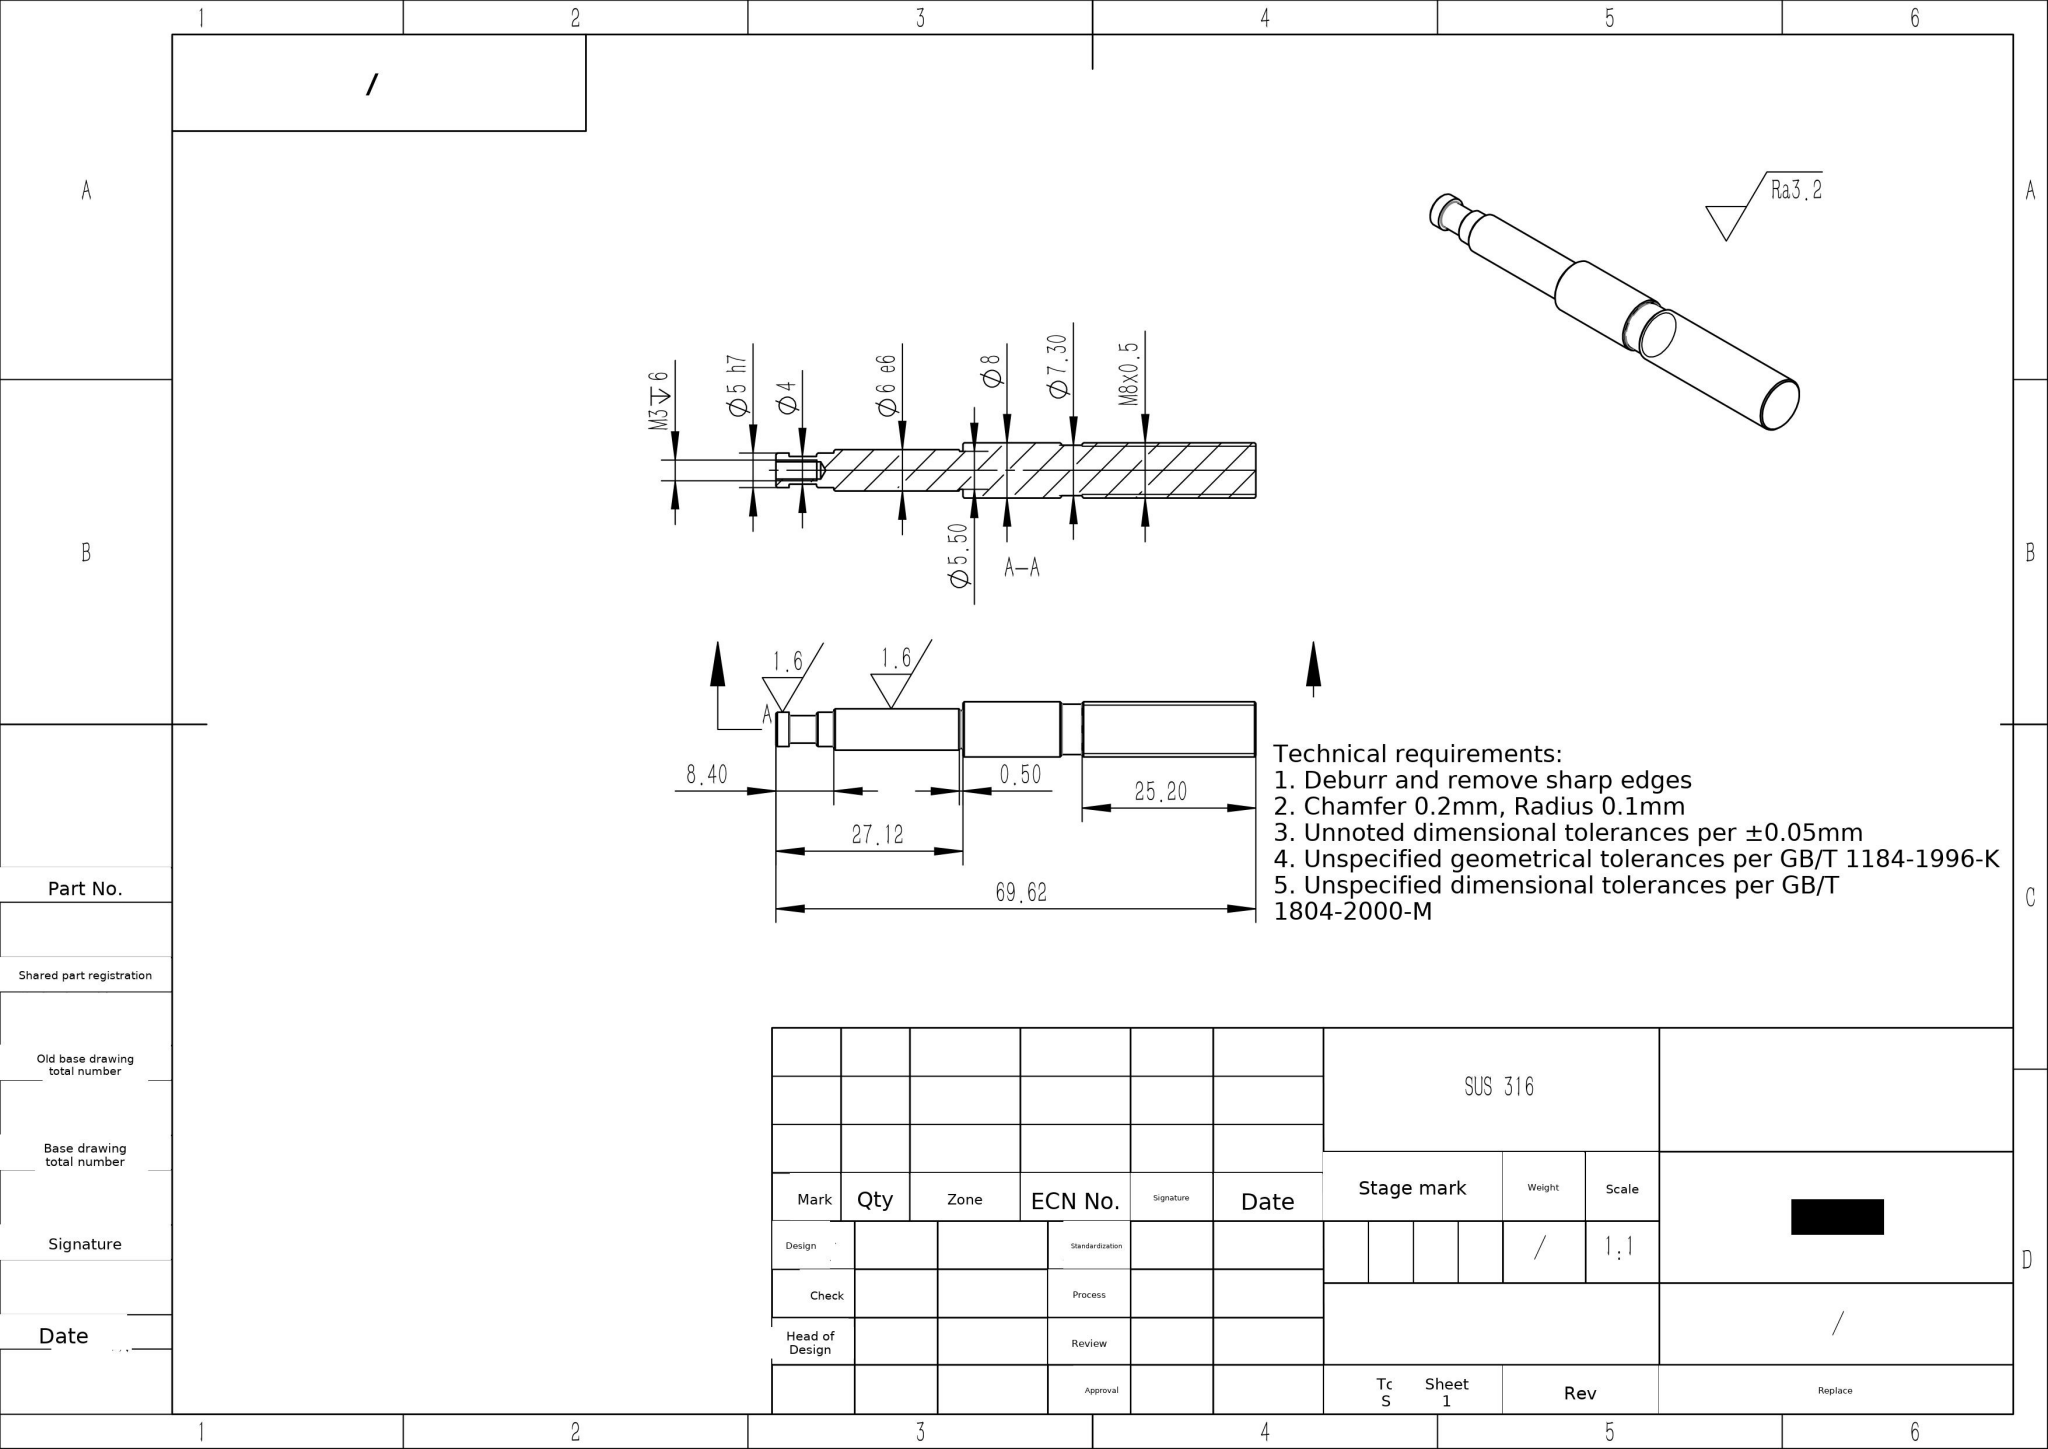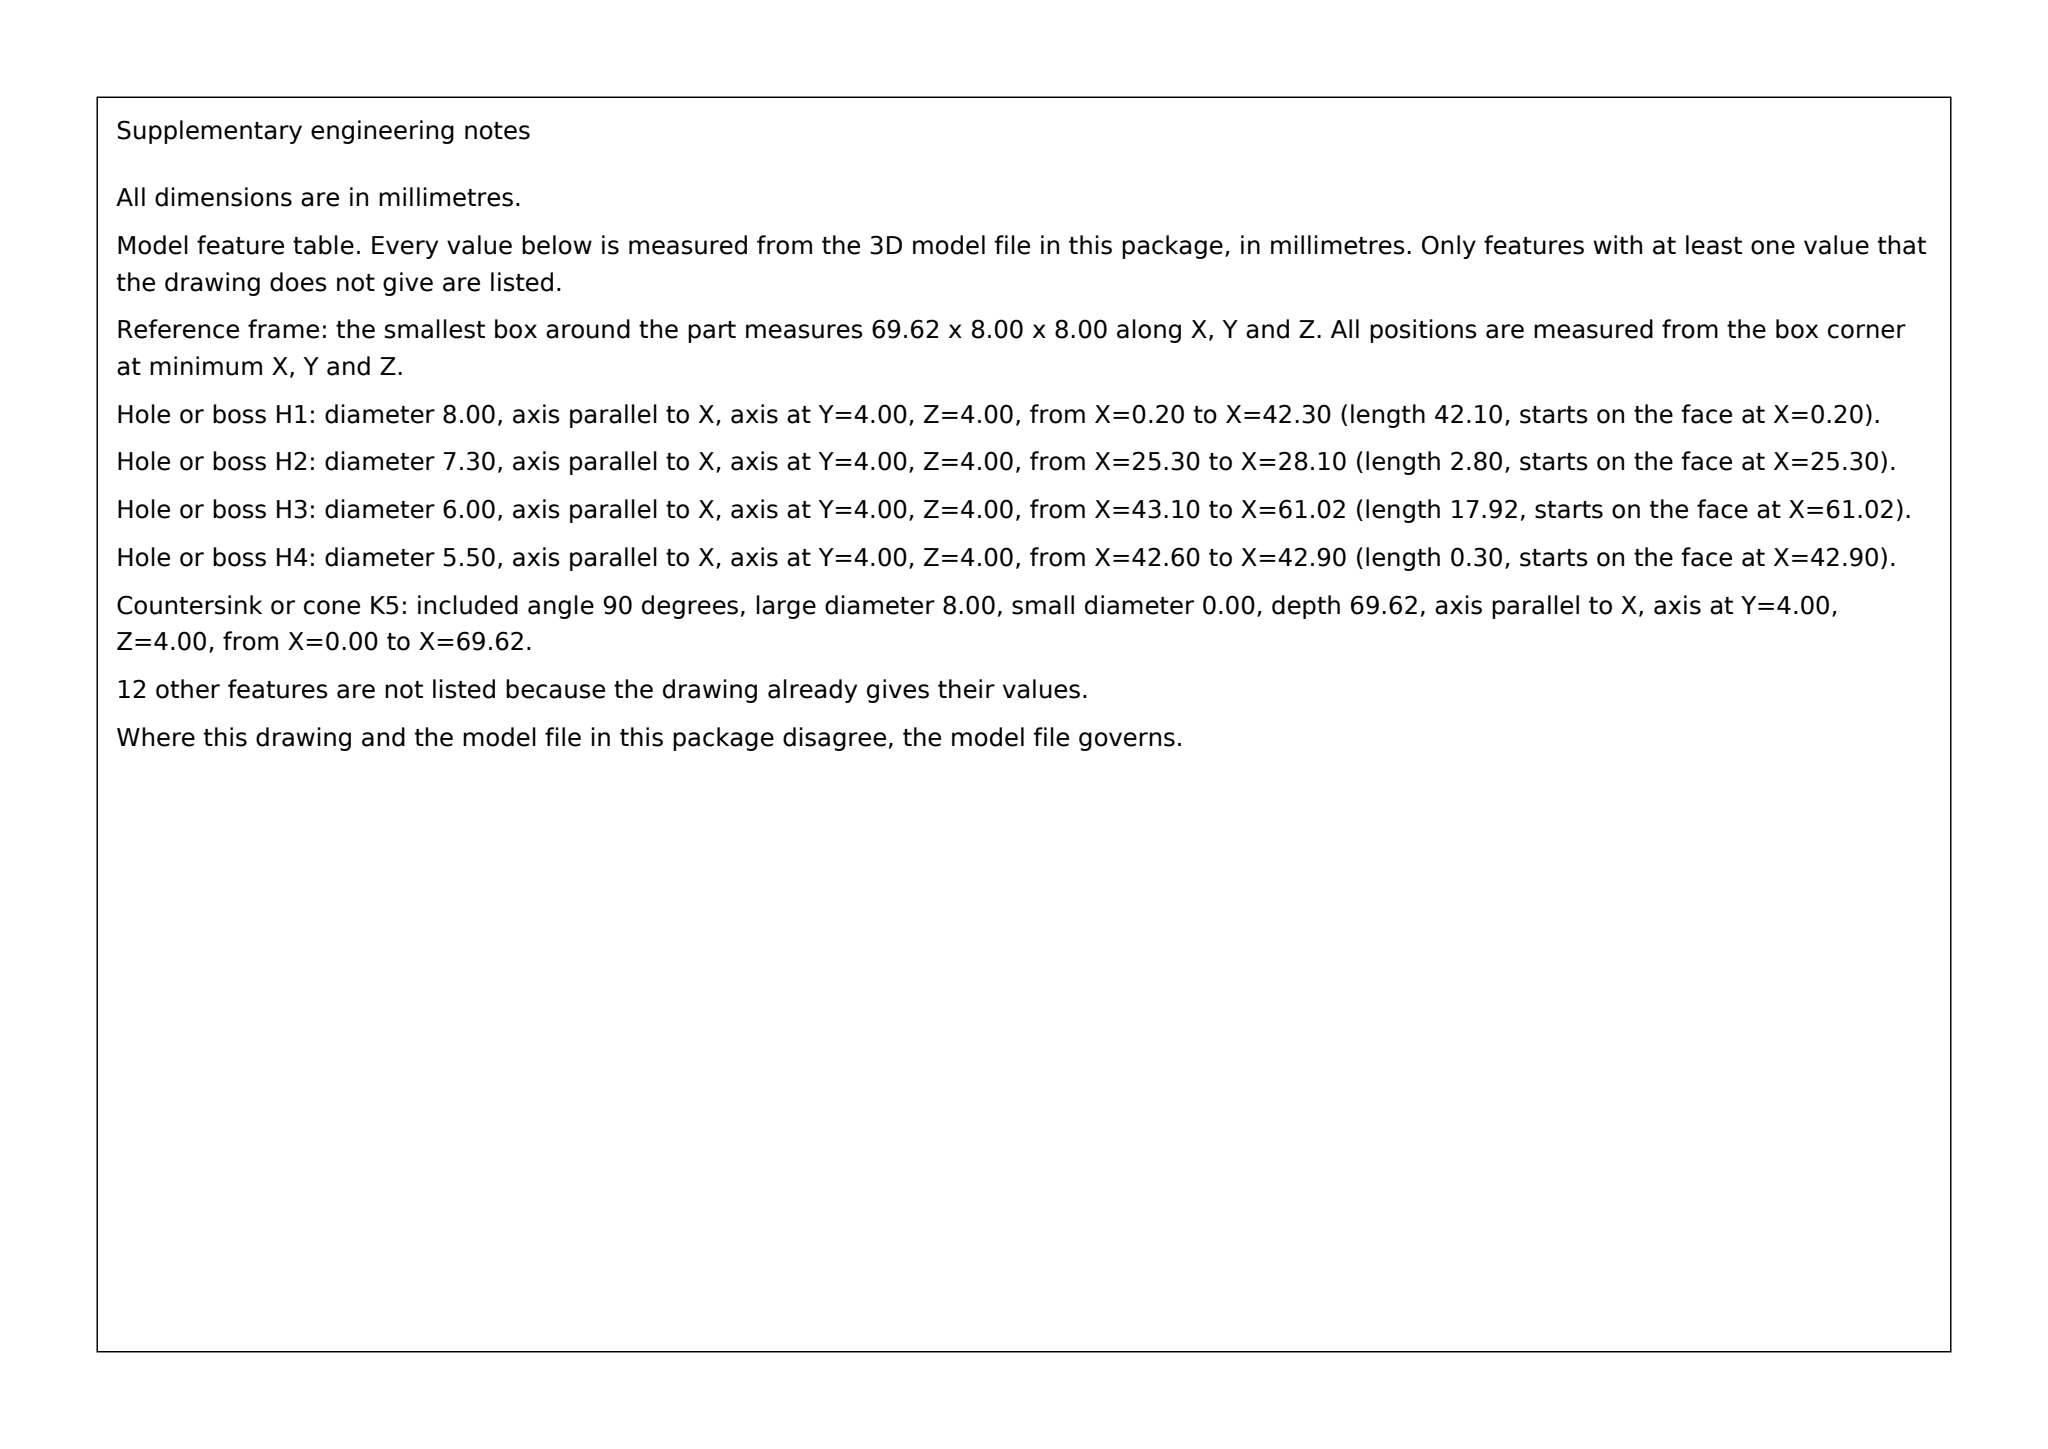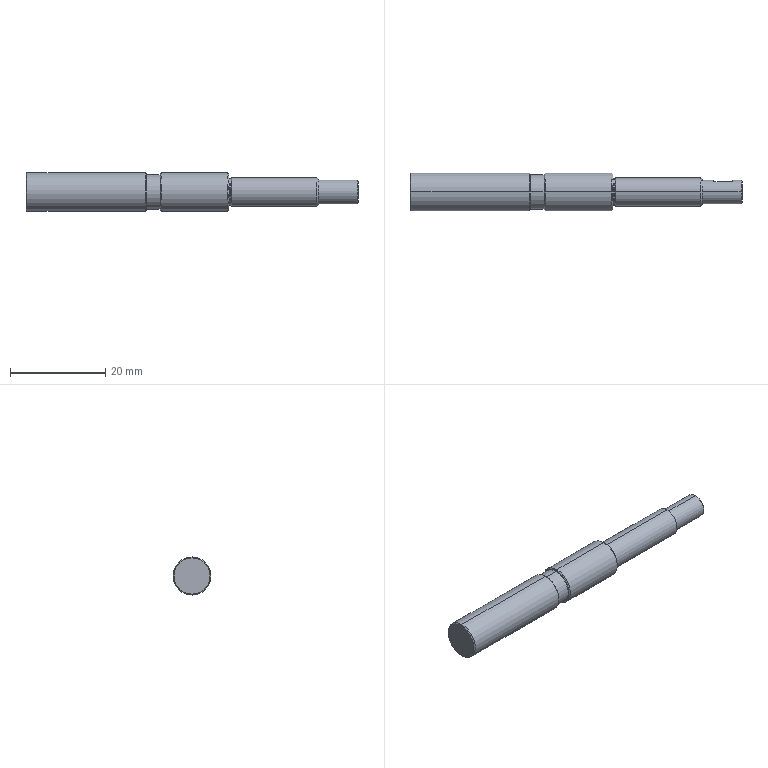Part | SolidWorks | mm | material SUS 316 | 1 solid | 50 faces | box 69.62 x 8 x 8 mm | volume 2764 mm3 | cone 16 | cylinder 14 | torus 10 | plane 10 | commonest cylinder face diameters 8 x4 5 x2 2.5 x2 6 x2 5.5 x2 7.3 x2